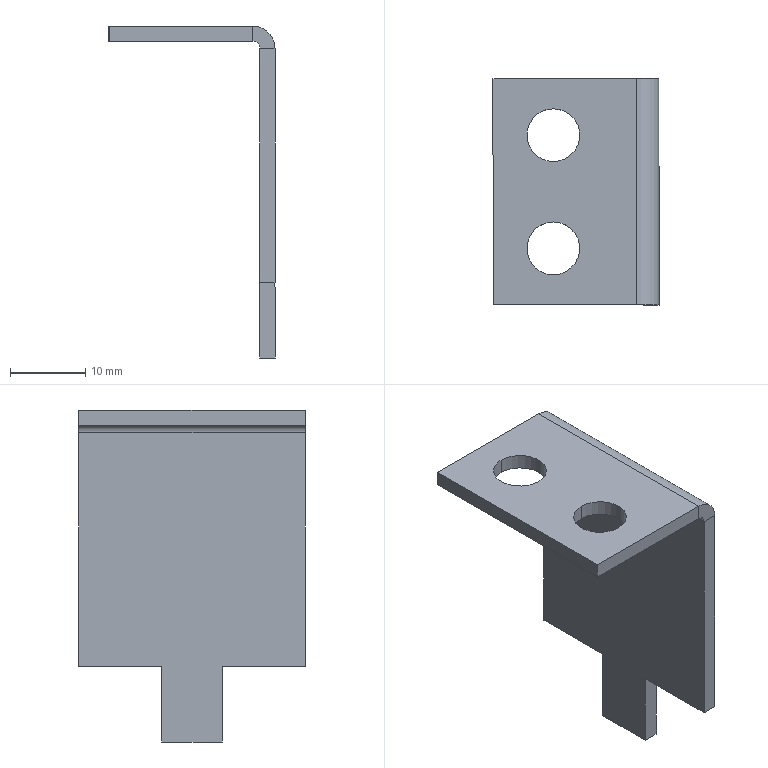Component | SolidWorks | 30-51A-1 | 1 solid | 22 faces | box 22 x 30 x 44 mm | volume 3195 mm3 | plane 16 | cylinder 6 | commonest cylinder face diameters 7 x4 2 x1 6 x1
STEP:
#1=CARTESIAN_POINT('',(-17.685,-3.193,0.9523));
#2=VERTEX_POINT('',#1);
#3=CARTESIAN_POINT('',(-17.685,-3.468,0.9523));
#4=VERTEX_POINT('',#3);
#5=CARTESIAN_POINT('',(-17.685,-3.33,0.9523));
#6=DIRECTION('',(0.,-0.,-1.));
#7=DIRECTION('',(0.,1.,0.));
#8=AXIS2_PLACEMENT_3D('',#5,#6,#7);
#9=CIRCLE('',#8,0.1378);
#10=EDGE_CURVE('',#2,#4,#9,.T.);
#11=ORIENTED_EDGE('',*,*,#10,.F.);
#12=CARTESIAN_POINT('',(-17.685,-3.193,0.8735));
#13=VERTEX_POINT('',#12);
#14=CARTESIAN_POINT('',(-17.685,-3.193,0.9523));
#15=DIRECTION('',(0.,-0.,-1.));
#16=VECTOR('',#15,39.37);
#17=LINE('',#14,#16);
#18=EDGE_CURVE('',#2,#13,#17,.T.);
#19=ORIENTED_EDGE('',*,*,#18,.T.);
#20=CARTESIAN_POINT('',(-17.685,-3.468,0.8735));
#21=VERTEX_POINT('',#20);
#22=CARTESIAN_POINT('',(-17.685,-3.33,0.8735));
#23=DIRECTION('',(0.,-0.,-1.));
#24=DIRECTION('',(0.,1.,0.));
#25=AXIS2_PLACEMENT_3D('',#22,#23,#24);
#26=CIRCLE('',#25,0.1378);
#27=EDGE_CURVE('',#13,#21,#26,.T.);
#28=ORIENTED_EDGE('',*,*,#27,.T.);
#29=CARTESIAN_POINT('',(-17.685,-3.468,0.9523));
#30=DIRECTION('',(0.,-0.,-1.));
#31=VECTOR('',#30,39.37);
#32=LINE('',#29,#31);
#33=EDGE_CURVE('',#4,#21,#32,.T.);
#34=ORIENTED_EDGE('',*,*,#33,.F.);
#35=EDGE_LOOP('',(#11,#19,#28,#34));
#36=FACE_OUTER_BOUND('',#35,.T.);
#37=CARTESIAN_POINT('',(-17.685,-3.33,0.9523));
#38=DIRECTION('',(0.,-0.,-1.));
#39=DIRECTION('',(0.,-1.,0.));
#40=AXIS2_PLACEMENT_3D('',#37,#38,#39);
#41=CYLINDRICAL_SURFACE('',#40,0.1378);
#42=ADVANCED_FACE('',(#36),#41,.F.);
#43=CARTESIAN_POINT('',(-17.685,-2.602,0.9523));
#44=VERTEX_POINT('',#43);
#45=CARTESIAN_POINT('',(-17.685,-2.878,0.9523));
#46=VERTEX_POINT('',#45);
#47=CARTESIAN_POINT('',(-17.685,-2.74,0.9523));
#48=DIRECTION('',(0.,-0.,-1.));
#49=DIRECTION('',(0.,-1.,0.));
#50=AXIS2_PLACEMENT_3D('',#47,#48,#49);
#51=CIRCLE('',#50,0.1378);
#52=EDGE_CURVE('',#44,#46,#51,.T.);
#53=ORIENTED_EDGE('',*,*,#52,.F.);
#54=CARTESIAN_POINT('',(-17.685,-2.602,0.8735));
#55=VERTEX_POINT('',#54);
#56=CARTESIAN_POINT('',(-17.685,-2.602,0.9523));
#57=DIRECTION('',(0.,-0.,-1.));
#58=VECTOR('',#57,39.37);
#59=LINE('',#56,#58);
#60=EDGE_CURVE('',#44,#55,#59,.T.);
#61=ORIENTED_EDGE('',*,*,#60,.T.);
#62=CARTESIAN_POINT('',(-17.685,-2.878,0.8735));
#63=VERTEX_POINT('',#62);
#64=CARTESIAN_POINT('',(-17.685,-2.74,0.8735));
#65=DIRECTION('',(0.,-0.,-1.));
#66=DIRECTION('',(0.,-1.,0.));
#67=AXIS2_PLACEMENT_3D('',#64,#65,#66);
#68=CIRCLE('',#67,0.1378);
#69=EDGE_CURVE('',#55,#63,#68,.T.);
#70=ORIENTED_EDGE('',*,*,#69,.T.);
#71=CARTESIAN_POINT('',(-17.685,-2.878,0.9523));
#72=DIRECTION('',(0.,-0.,-1.));
#73=VECTOR('',#72,39.37);
#74=LINE('',#71,#73);
#75=EDGE_CURVE('',#46,#63,#74,.T.);
#76=ORIENTED_EDGE('',*,*,#75,.F.);
#77=EDGE_LOOP('',(#53,#61,#70,#76));
#78=FACE_OUTER_BOUND('',#77,.T.);
#79=CARTESIAN_POINT('',(-17.685,-2.74,0.9523));
#80=DIRECTION('',(0.,-0.,-1.));
#81=DIRECTION('',(0.,-1.,0.));
#82=AXIS2_PLACEMENT_3D('',#79,#80,#81);
#83=CYLINDRICAL_SURFACE('',#82,0.1378);
#84=ADVANCED_FACE('',(#78),#83,.F.);
#85=CARTESIAN_POINT('',(-17.134,-3.626,-0.3863));
#86=VERTEX_POINT('',#85);
#87=CARTESIAN_POINT('',(-17.213,-3.626,-0.3863));
#88=VERTEX_POINT('',#87);
#89=CARTESIAN_POINT('',(-17.252,-3.626,-0.3863));
#90=DIRECTION('',(-1.,-0.,-0.));
#91=VECTOR('',#90,39.37);
#92=LINE('',#89,#91);
#93=EDGE_CURVE('',#86,#88,#92,.T.);
#94=ORIENTED_EDGE('',*,*,#93,.F.);
#95=CARTESIAN_POINT('',(-17.134,-3.626,0.8342));
#96=VERTEX_POINT('',#95);
#97=CARTESIAN_POINT('',(-17.134,-3.626,-0.78));
#98=DIRECTION('',(-0.,0.,1.));
#99=VECTOR('',#98,39.37);
#100=LINE('',#97,#99);
#101=EDGE_CURVE('',#86,#96,#100,.T.);
#102=ORIENTED_EDGE('',*,*,#101,.T.);
#103=CARTESIAN_POINT('',(-17.213,-3.626,0.8342));
#104=VERTEX_POINT('',#103);
#105=CARTESIAN_POINT('',(-17.134,-3.626,0.8342));
#106=DIRECTION('',(-1.,-0.,0.));
#107=VECTOR('',#106,39.37);
#108=LINE('',#105,#107);
#109=EDGE_CURVE('',#96,#104,#108,.T.);
#110=ORIENTED_EDGE('',*,*,#109,.T.);
#111=CARTESIAN_POINT('',(-17.213,-3.626,-0.78));
#112=DIRECTION('',(-0.,0.,1.));
#113=VECTOR('',#112,39.37);
#114=LINE('',#111,#113);
#115=EDGE_CURVE('',#88,#104,#114,.T.);
#116=ORIENTED_EDGE('',*,*,#115,.F.);
#117=EDGE_LOOP('',(#94,#102,#110,#116));
#118=FACE_OUTER_BOUND('',#117,.T.);
#119=CARTESIAN_POINT('',(-17.252,-3.626,0.8342));
#120=DIRECTION('',(-0.,1.,-0.));
#121=DIRECTION('',(1.,0.,0.));
#122=AXIS2_PLACEMENT_3D('',#119,#120,#121);
#123=PLANE('',#122);
#124=ADVANCED_FACE('',(#118),#123,.F.);
#125=CARTESIAN_POINT('',(-17.134,-2.445,-0.3863));
#126=VERTEX_POINT('',#125);
#127=CARTESIAN_POINT('',(-17.134,-2.445,0.8342));
#128=VERTEX_POINT('',#127);
#129=CARTESIAN_POINT('',(-17.134,-2.445,-0.78));
#130=DIRECTION('',(-0.,0.,1.));
#131=VECTOR('',#130,39.37);
#132=LINE('',#129,#131);
#133=EDGE_CURVE('',#126,#128,#132,.T.);
#134=ORIENTED_EDGE('',*,*,#133,.F.);
#135=CARTESIAN_POINT('',(-17.213,-2.445,-0.3863));
#136=VERTEX_POINT('',#135);
#137=CARTESIAN_POINT('',(-16.819,-2.445,-0.3863));
#138=DIRECTION('',(1.,0.,0.));
#139=VECTOR('',#138,39.37);
#140=LINE('',#137,#139);
#141=EDGE_CURVE('',#136,#126,#140,.T.);
#142=ORIENTED_EDGE('',*,*,#141,.F.);
#143=CARTESIAN_POINT('',(-17.213,-2.445,0.8342));
#144=VERTEX_POINT('',#143);
#145=CARTESIAN_POINT('',(-17.213,-2.445,-0.78));
#146=DIRECTION('',(-0.,0.,1.));
#147=VECTOR('',#146,39.37);
#148=LINE('',#145,#147);
#149=EDGE_CURVE('',#136,#144,#148,.T.);
#150=ORIENTED_EDGE('',*,*,#149,.T.);
#151=CARTESIAN_POINT('',(-17.213,-2.445,0.8342));
#152=DIRECTION('',(1.,0.,-0.));
#153=VECTOR('',#152,39.37);
#154=LINE('',#151,#153);
#155=EDGE_CURVE('',#144,#128,#154,.T.);
#156=ORIENTED_EDGE('',*,*,#155,.T.);
#157=EDGE_LOOP('',(#134,#142,#150,#156));
#158=FACE_OUTER_BOUND('',#157,.T.);
#159=CARTESIAN_POINT('',(-17.252,-2.445,0.9523));
#160=DIRECTION('',(-0.,1.,-0.));
#161=DIRECTION('',(1.,0.,0.));
#162=AXIS2_PLACEMENT_3D('',#159,#160,#161);
#163=PLANE('',#162);
#164=ADVANCED_FACE('',(#158),#163,.T.);
#165=CARTESIAN_POINT('',(-17.252,-3.626,0.8735));
#166=VERTEX_POINT('',#165);
#167=CARTESIAN_POINT('',(-17.252,-3.626,0.9523));
#168=VERTEX_POINT('',#167);
#169=CARTESIAN_POINT('',(-17.252,-3.626,0.8735));
#170=DIRECTION('',(-0.,0.,1.));
#171=VECTOR('',#170,39.37);
#172=LINE('',#169,#171);
#173=EDGE_CURVE('',#166,#168,#172,.T.);
#174=ORIENTED_EDGE('',*,*,#173,.F.);
#175=CARTESIAN_POINT('',(-17.252,-3.626,0.8342));
#176=DIRECTION('',(0.,-1.,0.));
#177=DIRECTION('',(1.,0.,0.));
#178=AXIS2_PLACEMENT_3D('',#175,#176,#177);
#179=CIRCLE('',#178,0.03937);
#180=EDGE_CURVE('',#104,#166,#179,.T.);
#181=ORIENTED_EDGE('',*,*,#180,.F.);
#182=ORIENTED_EDGE('',*,*,#109,.F.);
#183=CARTESIAN_POINT('',(-17.252,-3.626,0.8342));
#184=DIRECTION('',(0.,-1.,0.));
#185=DIRECTION('',(-1.,-0.,0.));
#186=AXIS2_PLACEMENT_3D('',#183,#184,#185);
#187=CIRCLE('',#186,0.1181);
#188=EDGE_CURVE('',#96,#168,#187,.T.);
#189=ORIENTED_EDGE('',*,*,#188,.T.);
#190=EDGE_LOOP('',(#174,#181,#182,#189));
#191=FACE_OUTER_BOUND('',#190,.T.);
#192=CARTESIAN_POINT('',(-17.252,-3.626,0.8735));
#193=DIRECTION('',(0.,-1.,0.));
#194=DIRECTION('',(-1.,-0.,-0.));
#195=AXIS2_PLACEMENT_3D('',#192,#193,#194);
#196=PLANE('',#195);
#197=ADVANCED_FACE('',(#191),#196,.T.);
#198=CARTESIAN_POINT('',(-18.,-3.626,0.8735));
#199=VERTEX_POINT('',#198);
#200=CARTESIAN_POINT('',(-17.213,-3.626,0.8735));
#201=DIRECTION('',(-1.,-0.,-0.));
#202=VECTOR('',#201,39.37);
#203=LINE('',#200,#202);
#204=EDGE_CURVE('',#166,#199,#203,.T.);
#205=ORIENTED_EDGE('',*,*,#204,.F.);
#206=ORIENTED_EDGE('',*,*,#173,.T.);
#207=CARTESIAN_POINT('',(-18.,-3.626,0.9523));
#208=VERTEX_POINT('',#207);
#209=CARTESIAN_POINT('',(-17.213,-3.626,0.9523));
#210=DIRECTION('',(-1.,-0.,-0.));
#211=VECTOR('',#210,39.37);
#212=LINE('',#209,#211);
#213=EDGE_CURVE('',#168,#208,#212,.T.);
#214=ORIENTED_EDGE('',*,*,#213,.T.);
#215=CARTESIAN_POINT('',(-18.,-3.626,0.8735));
#216=DIRECTION('',(-0.,0.,1.));
#217=VECTOR('',#216,39.37);
#218=LINE('',#215,#217);
#219=EDGE_CURVE('',#199,#208,#218,.T.);
#220=ORIENTED_EDGE('',*,*,#219,.F.);
#221=EDGE_LOOP('',(#205,#206,#214,#220));
#222=FACE_OUTER_BOUND('',#221,.T.);
#223=CARTESIAN_POINT('',(-17.134,-3.626,0.8342));
#224=DIRECTION('',(0.,-1.,0.));
#225=DIRECTION('',(-1.,-0.,-0.));
#226=AXIS2_PLACEMENT_3D('',#223,#224,#225);
#227=PLANE('',#226);
#228=ADVANCED_FACE('',(#222),#227,.T.);
#229=ORIENTED_EDGE('',*,*,#155,.F.);
#230=CARTESIAN_POINT('',(-17.252,-2.445,0.8735));
#231=VERTEX_POINT('',#230);
#232=CARTESIAN_POINT('',(-17.252,-2.445,0.8342));
#233=DIRECTION('',(0.,-1.,0.));
#234=DIRECTION('',(1.,0.,0.));
#235=AXIS2_PLACEMENT_3D('',#232,#233,#234);
#236=CIRCLE('',#235,0.03937);
#237=EDGE_CURVE('',#144,#231,#236,.T.);
#238=ORIENTED_EDGE('',*,*,#237,.T.);
#239=CARTESIAN_POINT('',(-17.252,-2.445,0.9523));
#240=VERTEX_POINT('',#239);
#241=CARTESIAN_POINT('',(-17.252,-2.445,0.9523));
#242=DIRECTION('',(0.,-0.,-1.));
#243=VECTOR('',#242,39.37);
#244=LINE('',#241,#243);
#245=EDGE_CURVE('',#240,#231,#244,.T.);
#246=ORIENTED_EDGE('',*,*,#245,.F.);
#247=CARTESIAN_POINT('',(-17.252,-2.445,0.8342));
#248=DIRECTION('',(0.,-1.,0.));
#249=DIRECTION('',(-1.,-0.,0.));
#250=AXIS2_PLACEMENT_3D('',#247,#248,#249);
#251=CIRCLE('',#250,0.1181);
#252=EDGE_CURVE('',#128,#240,#251,.T.);
#253=ORIENTED_EDGE('',*,*,#252,.F.);
#254=EDGE_LOOP('',(#229,#238,#246,#253));
#255=FACE_OUTER_BOUND('',#254,.T.);
#256=CARTESIAN_POINT('',(-17.213,-2.445,0.8342));
#257=DIRECTION('',(-0.,1.,-0.));
#258=DIRECTION('',(1.,0.,0.));
#259=AXIS2_PLACEMENT_3D('',#256,#257,#258);
#260=PLANE('',#259);
#261=ADVANCED_FACE('',(#255),#260,.T.);
#262=CARTESIAN_POINT('',(-17.685,-3.33,0.9523));
#263=DIRECTION('',(0.,-0.,-1.));
#264=DIRECTION('',(0.,1.,0.));
#265=AXIS2_PLACEMENT_3D('',#262,#263,#264);
#266=CIRCLE('',#265,0.1378);
#267=EDGE_CURVE('',#4,#2,#266,.T.);
#268=ORIENTED_EDGE('',*,*,#267,.T.);
#269=ORIENTED_EDGE('',*,*,#10,.T.);
#270=EDGE_LOOP('',(#268,#269));
#271=FACE_BOUND('',#270,.T.);
#272=CARTESIAN_POINT('',(-17.685,-2.74,0.9523));
#273=DIRECTION('',(0.,-0.,-1.));
#274=DIRECTION('',(0.,-1.,0.));
#275=AXIS2_PLACEMENT_3D('',#272,#273,#274);
#276=CIRCLE('',#275,0.1378);
#277=EDGE_CURVE('',#46,#44,#276,.T.);
#278=ORIENTED_EDGE('',*,*,#277,.T.);
#279=ORIENTED_EDGE('',*,*,#52,.T.);
#280=EDGE_LOOP('',(#278,#279));
#281=FACE_BOUND('',#280,.T.);
#282=CARTESIAN_POINT('',(-18.,-2.445,0.9523));
#283=VERTEX_POINT('',#282);
#284=CARTESIAN_POINT('',(-17.213,-2.445,0.9523));
#285=DIRECTION('',(-1.,-0.,-0.));
#286=VECTOR('',#285,39.37);
#287=LINE('',#284,#286);
#288=EDGE_CURVE('',#240,#283,#287,.T.);
#289=ORIENTED_EDGE('',*,*,#288,.T.);
#290=CARTESIAN_POINT('',(-18.,-3.626,0.9523));
#291=DIRECTION('',(-0.,1.,-0.));
#292=VECTOR('',#291,39.37);
#293=LINE('',#290,#292);
#294=EDGE_CURVE('',#208,#283,#293,.T.);
#295=ORIENTED_EDGE('',*,*,#294,.F.);
#296=ORIENTED_EDGE('',*,*,#213,.F.);
#297=CARTESIAN_POINT('',(-17.252,-3.626,0.9523));
#298=DIRECTION('',(-0.,1.,-0.));
#299=VECTOR('',#298,39.37);
#300=LINE('',#297,#299);
#301=EDGE_CURVE('',#168,#240,#300,.T.);
#302=ORIENTED_EDGE('',*,*,#301,.T.);
#303=EDGE_LOOP('',(#289,#295,#296,#302));
#304=FACE_OUTER_BOUND('',#303,.T.);
#305=CARTESIAN_POINT('',(-17.213,-3.626,0.9523));
#306=DIRECTION('',(0.,-0.,-1.));
#307=DIRECTION('',(0.,-1.,0.));
#308=AXIS2_PLACEMENT_3D('',#305,#306,#307);
#309=PLANE('',#308);
#310=ADVANCED_FACE('',(#271,#281,#304),#309,.F.);
#311=CARTESIAN_POINT('',(-18.,-2.445,0.8735));
#312=VERTEX_POINT('',#311);
#313=CARTESIAN_POINT('',(-18.,-2.445,0.8735));
#314=DIRECTION('',(-0.,0.,1.));
#315=VECTOR('',#314,39.37);
#316=LINE('',#313,#315);
#317=EDGE_CURVE('',#312,#283,#316,.T.);
#318=ORIENTED_EDGE('',*,*,#317,.F.);
#319=CARTESIAN_POINT('',(-18.,-3.626,0.8735));
#320=DIRECTION('',(-0.,1.,-0.));
#321=VECTOR('',#320,39.37);
#322=LINE('',#319,#321);
#323=EDGE_CURVE('',#199,#312,#322,.T.);
#324=ORIENTED_EDGE('',*,*,#323,.F.);
#325=ORIENTED_EDGE('',*,*,#219,.T.);
#326=ORIENTED_EDGE('',*,*,#294,.T.);
#327=EDGE_LOOP('',(#318,#324,#325,#326));
#328=FACE_OUTER_BOUND('',#327,.T.);
#329=CARTESIAN_POINT('',(-18.,-3.626,0.8735));
#330=DIRECTION('',(-1.,-0.,-0.));
#331=DIRECTION('',(-0.,1.,-0.));
#332=AXIS2_PLACEMENT_3D('',#329,#330,#331);
#333=PLANE('',#332);
#334=ADVANCED_FACE('',(#328),#333,.T.);
#335=CARTESIAN_POINT('',(-17.685,-3.33,0.8735));
#336=DIRECTION('',(0.,-0.,-1.));
#337=DIRECTION('',(0.,1.,0.));
#338=AXIS2_PLACEMENT_3D('',#335,#336,#337);
#339=CIRCLE('',#338,0.1378);
#340=EDGE_CURVE('',#21,#13,#339,.T.);
#341=ORIENTED_EDGE('',*,*,#340,.F.);
#342=ORIENTED_EDGE('',*,*,#27,.F.);
#343=EDGE_LOOP('',(#341,#342));
#344=FACE_BOUND('',#343,.T.);
#345=CARTESIAN_POINT('',(-17.685,-2.74,0.8735));
#346=DIRECTION('',(0.,-0.,-1.));
#347=DIRECTION('',(0.,-1.,0.));
#348=AXIS2_PLACEMENT_3D('',#345,#346,#347);
#349=CIRCLE('',#348,0.1378);
#350=EDGE_CURVE('',#63,#55,#349,.T.);
#351=ORIENTED_EDGE('',*,*,#350,.F.);
#352=ORIENTED_EDGE('',*,*,#69,.F.);
#353=EDGE_LOOP('',(#351,#352));
#354=FACE_BOUND('',#353,.T.);
#355=CARTESIAN_POINT('',(-17.213,-2.445,0.8735));
#356=DIRECTION('',(-1.,-0.,-0.));
#357=VECTOR('',#356,39.37);
#358=LINE('',#355,#357);
#359=EDGE_CURVE('',#231,#312,#358,.T.);
#360=ORIENTED_EDGE('',*,*,#359,.F.);
#361=CARTESIAN_POINT('',(-17.252,-3.626,0.8735));
#362=DIRECTION('',(-0.,1.,-0.));
#363=VECTOR('',#362,39.37);
#364=LINE('',#361,#363);
#365=EDGE_CURVE('',#166,#231,#364,.T.);
#366=ORIENTED_EDGE('',*,*,#365,.F.);
#367=ORIENTED_EDGE('',*,*,#204,.T.);
#368=ORIENTED_EDGE('',*,*,#323,.T.);
#369=EDGE_LOOP('',(#360,#366,#367,#368));
#370=FACE_OUTER_BOUND('',#369,.T.);
#371=CARTESIAN_POINT('',(-17.213,-3.626,0.8735));
#372=DIRECTION('',(0.,-0.,-1.));
#373=DIRECTION('',(0.,-1.,0.));
#374=AXIS2_PLACEMENT_3D('',#371,#372,#373);
#375=PLANE('',#374);
#376=ADVANCED_FACE('',(#344,#354,#370),#375,.T.);
#377=ORIENTED_EDGE('',*,*,#237,.F.);
#378=CARTESIAN_POINT('',(-17.213,-3.626,0.8342));
#379=DIRECTION('',(-0.,1.,-0.));
#380=VECTOR('',#379,39.37);
#381=LINE('',#378,#380);
#382=EDGE_CURVE('',#104,#144,#381,.T.);
#383=ORIENTED_EDGE('',*,*,#382,.F.);
#384=ORIENTED_EDGE('',*,*,#180,.T.);
#385=ORIENTED_EDGE('',*,*,#365,.T.);
#386=EDGE_LOOP('',(#377,#383,#384,#385));
#387=FACE_OUTER_BOUND('',#386,.T.);
#388=CARTESIAN_POINT('',(-17.252,-3.626,0.8342));
#389=DIRECTION('',(-0.,1.,-0.));
#390=DIRECTION('',(1.,0.,0.));
#391=AXIS2_PLACEMENT_3D('',#388,#389,#390);
#392=CYLINDRICAL_SURFACE('',#391,0.03937);
#393=ADVANCED_FACE('',(#387),#392,.F.);
#394=CARTESIAN_POINT('',(-17.213,-3.193,-0.3863));
#395=VERTEX_POINT('',#394);
#396=CARTESIAN_POINT('',(-17.213,-3.193,-0.78));
#397=VERTEX_POINT('',#396);
#398=CARTESIAN_POINT('',(-17.213,-3.193,-0.78));
#399=DIRECTION('',(0.,-0.,-1.));
#400=VECTOR('',#399,39.37);
#401=LINE('',#398,#400);
#402=EDGE_CURVE('',#395,#397,#401,.T.);
#403=ORIENTED_EDGE('',*,*,#402,.F.);
#404=CARTESIAN_POINT('',(-17.213,-3.626,-0.3863));
#405=DIRECTION('',(0.,-1.,0.));
#406=VECTOR('',#405,39.37);
#407=LINE('',#404,#406);
#408=EDGE_CURVE('',#395,#88,#407,.T.);
#409=ORIENTED_EDGE('',*,*,#408,.T.);
#410=ORIENTED_EDGE('',*,*,#115,.T.);
#411=ORIENTED_EDGE('',*,*,#382,.T.);
#412=ORIENTED_EDGE('',*,*,#149,.F.);
#413=CARTESIAN_POINT('',(-17.213,-2.878,-0.3863));
#414=VERTEX_POINT('',#413);
#415=CARTESIAN_POINT('',(-17.213,-3.626,-0.3863));
#416=DIRECTION('',(0.,-1.,0.));
#417=VECTOR('',#416,39.37);
#418=LINE('',#415,#417);
#419=EDGE_CURVE('',#136,#414,#418,.T.);
#420=ORIENTED_EDGE('',*,*,#419,.T.);
#421=CARTESIAN_POINT('',(-17.213,-2.878,-0.78));
#422=VERTEX_POINT('',#421);
#423=CARTESIAN_POINT('',(-17.213,-2.878,-0.78));
#424=DIRECTION('',(-0.,0.,1.));
#425=VECTOR('',#424,39.37);
#426=LINE('',#423,#425);
#427=EDGE_CURVE('',#422,#414,#426,.T.);
#428=ORIENTED_EDGE('',*,*,#427,.F.);
#429=CARTESIAN_POINT('',(-17.213,-3.626,-0.78));
#430=DIRECTION('',(-0.,1.,-0.));
#431=VECTOR('',#430,39.37);
#432=LINE('',#429,#431);
#433=EDGE_CURVE('',#397,#422,#432,.T.);
#434=ORIENTED_EDGE('',*,*,#433,.F.);
#435=EDGE_LOOP('',(#403,#409,#410,#411,#412,#420,#428,#434));
#436=FACE_OUTER_BOUND('',#435,.T.);
#437=CARTESIAN_POINT('',(-17.213,-3.626,-0.78));
#438=DIRECTION('',(-1.,-0.,-0.));
#439=DIRECTION('',(0.,-0.,-1.));
#440=AXIS2_PLACEMENT_3D('',#437,#438,#439);
#441=PLANE('',#440);
#442=ADVANCED_FACE('',(#436),#441,.T.);
#443=CARTESIAN_POINT('',(-17.134,-3.193,-0.78));
#444=VERTEX_POINT('',#443);
#445=CARTESIAN_POINT('',(-16.819,-3.193,-0.78));
#446=DIRECTION('',(1.,0.,0.));
#447=VECTOR('',#446,39.37);
#448=LINE('',#445,#447);
#449=EDGE_CURVE('',#397,#444,#448,.T.);
#450=ORIENTED_EDGE('',*,*,#449,.F.);
#451=ORIENTED_EDGE('',*,*,#433,.T.);
#452=CARTESIAN_POINT('',(-17.134,-2.878,-0.78));
#453=VERTEX_POINT('',#452);
#454=CARTESIAN_POINT('',(-16.819,-2.878,-0.78));
#455=DIRECTION('',(-1.,-0.,-0.));
#456=VECTOR('',#455,39.37);
#457=LINE('',#454,#456);
#458=EDGE_CURVE('',#453,#422,#457,.T.);
#459=ORIENTED_EDGE('',*,*,#458,.F.);
#460=CARTESIAN_POINT('',(-17.134,-3.626,-0.78));
#461=DIRECTION('',(-0.,1.,-0.));
#462=VECTOR('',#461,39.37);
#463=LINE('',#460,#462);
#464=EDGE_CURVE('',#444,#453,#463,.T.);
#465=ORIENTED_EDGE('',*,*,#464,.F.);
#466=EDGE_LOOP('',(#450,#451,#459,#465));
#467=FACE_OUTER_BOUND('',#466,.T.);
#468=CARTESIAN_POINT('',(-17.134,-3.626,-0.78));
#469=DIRECTION('',(0.,-0.,-1.));
#470=DIRECTION('',(0.,-1.,0.));
#471=AXIS2_PLACEMENT_3D('',#468,#469,#470);
#472=PLANE('',#471);
#473=ADVANCED_FACE('',(#467),#472,.T.);
#474=CARTESIAN_POINT('',(-17.134,-3.193,-0.3863));
#475=VERTEX_POINT('',#474);
#476=CARTESIAN_POINT('',(-17.134,-3.626,-0.3863));
#477=DIRECTION('',(0.,-1.,0.));
#478=VECTOR('',#477,39.37);
#479=LINE('',#476,#478);
#480=EDGE_CURVE('',#475,#86,#479,.T.);
#481=ORIENTED_EDGE('',*,*,#480,.F.);
#482=CARTESIAN_POINT('',(-17.134,-3.193,-0.78));
#483=DIRECTION('',(0.,-0.,-1.));
#484=VECTOR('',#483,39.37);
#485=LINE('',#482,#484);
#486=EDGE_CURVE('',#475,#444,#485,.T.);
#487=ORIENTED_EDGE('',*,*,#486,.T.);
#488=ORIENTED_EDGE('',*,*,#464,.T.);
#489=CARTESIAN_POINT('',(-17.134,-2.878,-0.3863));
#490=VERTEX_POINT('',#489);
#491=CARTESIAN_POINT('',(-17.134,-2.878,-0.78));
#492=DIRECTION('',(-0.,0.,1.));
#493=VECTOR('',#492,39.37);
#494=LINE('',#491,#493);
#495=EDGE_CURVE('',#453,#490,#494,.T.);
#496=ORIENTED_EDGE('',*,*,#495,.T.);
#497=CARTESIAN_POINT('',(-17.134,-3.626,-0.3863));
#498=DIRECTION('',(0.,-1.,0.));
#499=VECTOR('',#498,39.37);
#500=LINE('',#497,#499);
#501=EDGE_CURVE('',#126,#490,#500,.T.);
#502=ORIENTED_EDGE('',*,*,#501,.F.);
#503=ORIENTED_EDGE('',*,*,#133,.T.);
#504=CARTESIAN_POINT('',(-17.134,-3.626,0.8342));
#505=DIRECTION('',(-0.,1.,-0.));
#506=VECTOR('',#505,39.37);
#507=LINE('',#504,#506);
#508=EDGE_CURVE('',#96,#128,#507,.T.);
#509=ORIENTED_EDGE('',*,*,#508,.F.);
#510=ORIENTED_EDGE('',*,*,#101,.F.);
#511=EDGE_LOOP('',(#481,#487,#488,#496,#502,#503,#509,#510));
#512=FACE_OUTER_BOUND('',#511,.T.);
#513=CARTESIAN_POINT('',(-17.134,-3.626,-0.78));
#514=DIRECTION('',(-1.,-0.,-0.));
#515=DIRECTION('',(0.,-0.,-1.));
#516=AXIS2_PLACEMENT_3D('',#513,#514,#515);
#517=PLANE('',#516);
#518=ADVANCED_FACE('',(#512),#517,.F.);
#519=ORIENTED_EDGE('',*,*,#252,.T.);
#520=ORIENTED_EDGE('',*,*,#301,.F.);
#521=ORIENTED_EDGE('',*,*,#188,.F.);
#522=ORIENTED_EDGE('',*,*,#508,.T.);
#523=EDGE_LOOP('',(#519,#520,#521,#522));
#524=FACE_OUTER_BOUND('',#523,.T.);
#525=CARTESIAN_POINT('',(-17.252,-3.626,0.8342));
#526=DIRECTION('',(-0.,1.,-0.));
#527=DIRECTION('',(1.,0.,0.));
#528=AXIS2_PLACEMENT_3D('',#525,#526,#527);
#529=CYLINDRICAL_SURFACE('',#528,0.1181);
#530=ADVANCED_FACE('',(#524),#529,.T.);
#531=ORIENTED_EDGE('',*,*,#288,.F.);
#532=ORIENTED_EDGE('',*,*,#245,.T.);
#533=ORIENTED_EDGE('',*,*,#359,.T.);
#534=ORIENTED_EDGE('',*,*,#317,.T.);
#535=EDGE_LOOP('',(#531,#532,#533,#534));
#536=FACE_OUTER_BOUND('',#535,.T.);
#537=CARTESIAN_POINT('',(-17.252,-2.445,0.8342));
#538=DIRECTION('',(-0.,1.,-0.));
#539=DIRECTION('',(1.,0.,0.));
#540=AXIS2_PLACEMENT_3D('',#537,#538,#539);
#541=PLANE('',#540);
#542=ADVANCED_FACE('',(#536),#541,.T.);
#543=ORIENTED_EDGE('',*,*,#427,.T.);
#544=CARTESIAN_POINT('',(-16.819,-2.878,-0.3863));
#545=DIRECTION('',(-1.,-0.,-0.));
#546=VECTOR('',#545,39.37);
#547=LINE('',#544,#546);
#548=EDGE_CURVE('',#490,#414,#547,.T.);
#549=ORIENTED_EDGE('',*,*,#548,.F.);
#550=ORIENTED_EDGE('',*,*,#495,.F.);
#551=ORIENTED_EDGE('',*,*,#458,.T.);
#552=EDGE_LOOP('',(#543,#549,#550,#551));
#553=FACE_OUTER_BOUND('',#552,.T.);
#554=CARTESIAN_POINT('',(-16.819,-2.878,-0.3863));
#555=DIRECTION('',(0.,-1.,0.));
#556=DIRECTION('',(-1.,-0.,-0.));
#557=AXIS2_PLACEMENT_3D('',#554,#555,#556);
#558=PLANE('',#557);
#559=ADVANCED_FACE('',(#553),#558,.F.);
#560=ORIENTED_EDGE('',*,*,#141,.T.);
#561=ORIENTED_EDGE('',*,*,#501,.T.);
#562=ORIENTED_EDGE('',*,*,#548,.T.);
#563=ORIENTED_EDGE('',*,*,#419,.F.);
#564=EDGE_LOOP('',(#560,#561,#562,#563));
#565=FACE_OUTER_BOUND('',#564,.T.);
#566=CARTESIAN_POINT('',(-16.819,-2.878,-0.3863));
#567=DIRECTION('',(0.,-0.,-1.));
#568=DIRECTION('',(0.,-1.,0.));
#569=AXIS2_PLACEMENT_3D('',#566,#567,#568);
#570=PLANE('',#569);
#571=ADVANCED_FACE('',(#565),#570,.T.);
#572=ORIENTED_EDGE('',*,*,#402,.T.);
#573=ORIENTED_EDGE('',*,*,#449,.T.);
#574=ORIENTED_EDGE('',*,*,#486,.F.);
#575=CARTESIAN_POINT('',(-16.819,-3.193,-0.3863));
#576=DIRECTION('',(1.,0.,0.));
#577=VECTOR('',#576,39.37);
#578=LINE('',#575,#577);
#579=EDGE_CURVE('',#395,#475,#578,.T.);
#580=ORIENTED_EDGE('',*,*,#579,.F.);
#581=EDGE_LOOP('',(#572,#573,#574,#580));
#582=FACE_OUTER_BOUND('',#581,.T.);
#583=CARTESIAN_POINT('',(-16.819,-3.193,-0.3863));
#584=DIRECTION('',(-0.,1.,-0.));
#585=DIRECTION('',(1.,0.,0.));
#586=AXIS2_PLACEMENT_3D('',#583,#584,#585);
#587=PLANE('',#586);
#588=ADVANCED_FACE('',(#582),#587,.F.);
#589=ORIENTED_EDGE('',*,*,#579,.T.);
#590=ORIENTED_EDGE('',*,*,#480,.T.);
#591=ORIENTED_EDGE('',*,*,#93,.T.);
#592=ORIENTED_EDGE('',*,*,#408,.F.);
#593=EDGE_LOOP('',(#589,#590,#591,#592));
#594=FACE_OUTER_BOUND('',#593,.T.);
#595=CARTESIAN_POINT('',(-17.252,-3.626,-0.3863));
#596=DIRECTION('',(0.,-0.,-1.));
#597=DIRECTION('',(0.,-1.,0.));
#598=AXIS2_PLACEMENT_3D('',#595,#596,#597);
#599=PLANE('',#598);
#600=ADVANCED_FACE('',(#594),#599,.T.);
#601=ORIENTED_EDGE('',*,*,#60,.F.);
#602=ORIENTED_EDGE('',*,*,#277,.F.);
#603=ORIENTED_EDGE('',*,*,#75,.T.);
#604=ORIENTED_EDGE('',*,*,#350,.T.);
#605=EDGE_LOOP('',(#601,#602,#603,#604));
#606=FACE_OUTER_BOUND('',#605,.T.);
#607=CARTESIAN_POINT('',(-17.685,-2.74,0.9523));
#608=DIRECTION('',(0.,-0.,-1.));
#609=DIRECTION('',(0.,-1.,0.));
#610=AXIS2_PLACEMENT_3D('',#607,#608,#609);
#611=CYLINDRICAL_SURFACE('',#610,0.1378);
#612=ADVANCED_FACE('',(#606),#611,.F.);
#613=ORIENTED_EDGE('',*,*,#18,.F.);
#614=ORIENTED_EDGE('',*,*,#267,.F.);
#615=ORIENTED_EDGE('',*,*,#33,.T.);
#616=ORIENTED_EDGE('',*,*,#340,.T.);
#617=EDGE_LOOP('',(#613,#614,#615,#616));
#618=FACE_OUTER_BOUND('',#617,.T.);
#619=CARTESIAN_POINT('',(-17.685,-3.33,0.9523));
#620=DIRECTION('',(0.,-0.,-1.));
#621=DIRECTION('',(0.,-1.,0.));
#622=AXIS2_PLACEMENT_3D('',#619,#620,#621);
#623=CYLINDRICAL_SURFACE('',#622,0.1378);
#624=ADVANCED_FACE('',(#618),#623,.F.);
#625=CLOSED_SHELL('',(#42,#84,#124,#164,#197,#228,#261,#310,#334,#376,#393,#442,#473,#518,#530,#542,#559,#571,#588,#600,#612,#624));
#626=MANIFOLD_SOLID_BREP('',#625);
#627=CARTESIAN_POINT('',(0.,0.,0.));
#628=DIRECTION('',(0.,0.,1.));
#629=DIRECTION('',(1.,0.,0.));
#630=AXIS2_PLACEMENT_3D('',#627,#628,#629);
#631=(LENGTH_UNIT()NAMED_UNIT(*)SI_UNIT($,.METRE.));
#632=LENGTH_MEASURE_WITH_UNIT(LENGTH_MEASURE(0.0254),#631);
#633=DIMENSIONAL_EXPONENTS(1.,0.,0.,0.,0.,0.,0.);
#634=(CONVERSION_BASED_UNIT('',#632)LENGTH_UNIT()NAMED_UNIT(#633));
#635=UNCERTAINTY_MEASURE_WITH_UNIT(LENGTH_MEASURE(0.00001),#634,'','');
#636=(NAMED_UNIT(*)PLANE_ANGLE_UNIT()SI_UNIT($,.RADIAN.));
#637=(NAMED_UNIT(*)SI_UNIT($,.STERADIAN.)SOLID_ANGLE_UNIT());
#638=(GEOMETRIC_REPRESENTATION_CONTEXT(3)GLOBAL_UNCERTAINTY_ASSIGNED_CONTEXT((#635))GLOBAL_UNIT_ASSIGNED_CONTEXT((#634,#636,#637))REPRESENTATION_CONTEXT('',''));
#639=ADVANCED_BREP_SHAPE_REPRESENTATION('',(#626,#630),#638);
#640=COLOUR_RGB('',0.7922,0.8196,0.9333);
#641=FILL_AREA_STYLE_COLOUR('',#640);
#642=FILL_AREA_STYLE('',(#641));
#643=SURFACE_STYLE_FILL_AREA(#642);
#644=SURFACE_SIDE_STYLE('',(#643));
#645=SURFACE_STYLE_USAGE(.BOTH.,#644);
#646=PRESENTATION_STYLE_ASSIGNMENT((#645));
#647=STYLED_ITEM('',(#646),#626);
#648=(LENGTH_UNIT()NAMED_UNIT(*)SI_UNIT($,.METRE.));
#649=LENGTH_MEASURE_WITH_UNIT(LENGTH_MEASURE(0.0254),#648);
#650=DIMENSIONAL_EXPONENTS(1.,0.,0.,0.,0.,0.,0.);
#651=(CONVERSION_BASED_UNIT('',#649)LENGTH_UNIT()NAMED_UNIT(#650));
#652=UNCERTAINTY_MEASURE_WITH_UNIT(LENGTH_MEASURE(0.00001),#651,'','');
#653=(NAMED_UNIT(*)PLANE_ANGLE_UNIT()SI_UNIT($,.RADIAN.));
#654=(NAMED_UNIT(*)SI_UNIT($,.STERADIAN.)SOLID_ANGLE_UNIT());
#655=(GEOMETRIC_REPRESENTATION_CONTEXT(3)GLOBAL_UNCERTAINTY_ASSIGNED_CONTEXT((#652))GLOBAL_UNIT_ASSIGNED_CONTEXT((#651,#653,#654))REPRESENTATION_CONTEXT('',''));
#656=MECHANICAL_DESIGN_GEOMETRIC_PRESENTATION_REPRESENTATION('',(#647),#655);
#657=PRESENTATION_LAYER_ASSIGNMENT('','',(#647));